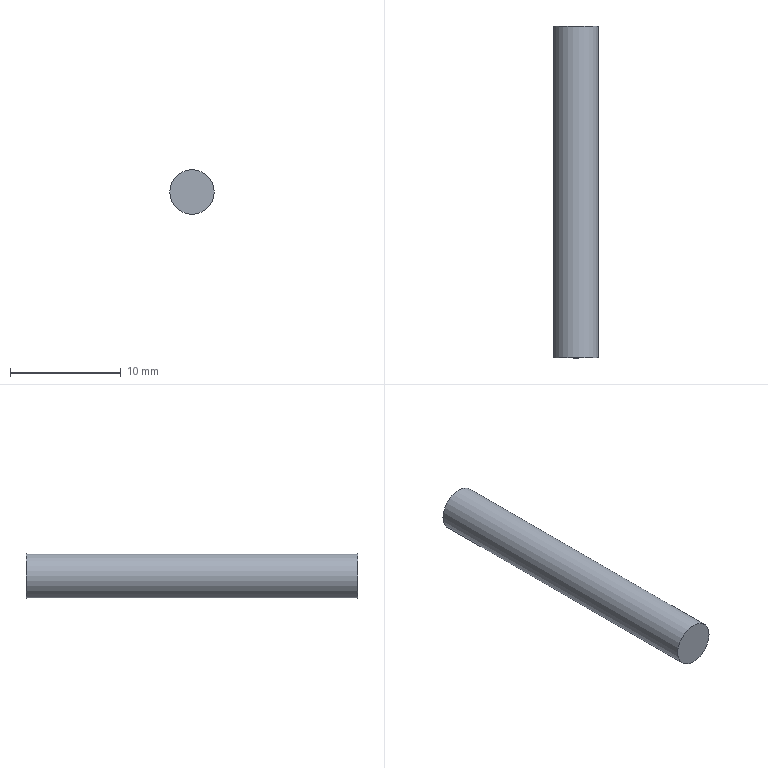Component | NX | STUD_M4 | 1 solid | 3 faces | box 4.01 x 30 x 4.01 mm | volume 379 mm3 | plane 2 | cylinder 1 | commonest cylinder face diameters 4.013 x1
STEP:
#1=CARTESIAN_POINT('',(0.,0.,0.));
#2=DIRECTION('',(0.,0.,1.));
#3=DIRECTION('',(1.,0.,0.));
#4=AXIS2_PLACEMENT_3D('',#1,#2,#3);
#5=CARTESIAN_POINT('',(-9.993,32.5,129.5));
#6=VERTEX_POINT('',#5);
#7=CARTESIAN_POINT('',(-12.,32.5,129.5));
#8=DIRECTION('',(0.,-1.,0.));
#9=DIRECTION('',(1.,0.,0.));
#10=AXIS2_PLACEMENT_3D('',#7,#8,#9);
#11=CIRCLE('',#10,2.007);
#12=CARTESIAN_POINT('',(-12.,32.5,129.5));
#13=DIRECTION('',(0.,1.,0.));
#14=DIRECTION('',(1.,0.,0.));
#15=AXIS2_PLACEMENT_3D('',#12,#13,#14);
#16=PLANE('',#15);
#17=CARTESIAN_POINT('',(2.007,0.));
#18=CARTESIAN_POINT('',(2.007,-3.476));
#19=CARTESIAN_POINT('',(-1.003,-1.738));
#20=CARTESIAN_POINT('',(-4.013,-0.));
#21=CARTESIAN_POINT('',(-1.003,1.738));
#22=CARTESIAN_POINT('',(2.007,3.476));
#23=CARTESIAN_POINT('',(2.007,0.));
#24=(BOUNDED_CURVE()B_SPLINE_CURVE(2,(#17,#18,#19,#20,#21,#22,#23),.UNSPECIFIED.,.T.,.F.)B_SPLINE_CURVE_WITH_KNOTS((1,2,2,2,2,1),(-2.094,0.,2.094,4.189,6.283,8.378),.UNSPECIFIED.)CURVE()GEOMETRIC_REPRESENTATION_ITEM()RATIONAL_B_SPLINE_CURVE((1.,0.5,1.,0.5,1.,0.5,1.))REPRESENTATION_ITEM(''));
#25=(GEOMETRIC_REPRESENTATION_CONTEXT(2)PARAMETRIC_REPRESENTATION_CONTEXT()REPRESENTATION_CONTEXT('',''));
#26=DEFINITIONAL_REPRESENTATION('',(#24),#25);
#27=PCURVE('',#16,#26);
#28=CARTESIAN_POINT('',(-12.,2.5,129.5));
#29=DIRECTION('',(0.,1.,0.));
#30=DIRECTION('',(1.,0.,0.));
#31=AXIS2_PLACEMENT_3D('',#28,#29,#30);
#32=CYLINDRICAL_SURFACE('',#31,2.007);
#33=CARTESIAN_POINT('',(6.283,30.));
#34=DIRECTION('',(-1.,0.));
#35=VECTOR('',#34,1.);
#36=LINE('',#33,#35);
#37=(GEOMETRIC_REPRESENTATION_CONTEXT(2)PARAMETRIC_REPRESENTATION_CONTEXT()REPRESENTATION_CONTEXT('',''));
#38=DEFINITIONAL_REPRESENTATION('',(#36),#37);
#39=PCURVE('',#32,#38);
#40=SURFACE_CURVE('',#11,(#27,#39),.PCURVE_S1.);
#41=EDGE_CURVE('',#6,#6,#40,.T.);
#42=ORIENTED_EDGE('',*,*,#41,.F.);
#43=EDGE_LOOP('',(#42));
#44=FACE_BOUND('',#43,.T.);
#45=ADVANCED_FACE('',(#44),#16,.T.);
#46=CARTESIAN_POINT('',(-9.993,2.5,129.5));
#47=VERTEX_POINT('',#46);
#48=CARTESIAN_POINT('',(-12.,2.5,129.5));
#49=DIRECTION('',(0.,1.,0.));
#50=DIRECTION('',(1.,0.,0.));
#51=AXIS2_PLACEMENT_3D('',#48,#49,#50);
#52=CIRCLE('',#51,2.007);
#53=CARTESIAN_POINT('',(-12.,2.5,129.5));
#54=DIRECTION('',(0.,-1.,0.));
#55=DIRECTION('',(-1.,0.,0.));
#56=AXIS2_PLACEMENT_3D('',#53,#54,#55);
#57=PLANE('',#56);
#58=CARTESIAN_POINT('',(-2.007,0.));
#59=CARTESIAN_POINT('',(-2.007,3.476));
#60=CARTESIAN_POINT('',(1.003,1.738));
#61=CARTESIAN_POINT('',(4.013,0.));
#62=CARTESIAN_POINT('',(1.003,-1.738));
#63=CARTESIAN_POINT('',(-2.007,-3.476));
#64=CARTESIAN_POINT('',(-2.007,0.));
#65=(BOUNDED_CURVE()B_SPLINE_CURVE(2,(#58,#59,#60,#61,#62,#63,#64),.UNSPECIFIED.,.T.,.F.)B_SPLINE_CURVE_WITH_KNOTS((1,2,2,2,2,1),(-2.094,0.,2.094,4.189,6.283,8.378),.UNSPECIFIED.)CURVE()GEOMETRIC_REPRESENTATION_ITEM()RATIONAL_B_SPLINE_CURVE((1.,0.5,1.,0.5,1.,0.5,1.))REPRESENTATION_ITEM(''));
#66=(GEOMETRIC_REPRESENTATION_CONTEXT(2)PARAMETRIC_REPRESENTATION_CONTEXT()REPRESENTATION_CONTEXT('',''));
#67=DEFINITIONAL_REPRESENTATION('',(#65),#66);
#68=PCURVE('',#57,#67);
#69=CARTESIAN_POINT('',(0.,0.));
#70=DIRECTION('',(1.,0.));
#71=VECTOR('',#70,1.);
#72=LINE('',#69,#71);
#73=(GEOMETRIC_REPRESENTATION_CONTEXT(2)PARAMETRIC_REPRESENTATION_CONTEXT()REPRESENTATION_CONTEXT('',''));
#74=DEFINITIONAL_REPRESENTATION('',(#72),#73);
#75=PCURVE('',#32,#74);
#76=SURFACE_CURVE('',#52,(#68,#75),.PCURVE_S1.);
#77=EDGE_CURVE('',#47,#47,#76,.T.);
#78=ORIENTED_EDGE('',*,*,#77,.F.);
#79=EDGE_LOOP('',(#78));
#80=FACE_BOUND('',#79,.T.);
#81=ADVANCED_FACE('',(#80),#57,.T.);
#82=ORIENTED_EDGE('',*,*,#41,.T.);
#83=CARTESIAN_POINT('',(-9.993,2.5,129.5));
#84=CARTESIAN_POINT('',(-9.993,32.5,129.5));
#85=B_SPLINE_CURVE_WITH_KNOTS('',1,(#83,#84),.UNSPECIFIED.,.F.,.F.,(2,2),(0.,30.),.PIECEWISE_BEZIER_KNOTS.);
#86=CARTESIAN_POINT('',(0.,0.));
#87=DIRECTION('',(0.,1.));
#88=VECTOR('',#87,1.);
#89=LINE('',#86,#88);
#90=(GEOMETRIC_REPRESENTATION_CONTEXT(2)PARAMETRIC_REPRESENTATION_CONTEXT()REPRESENTATION_CONTEXT('',''));
#91=DEFINITIONAL_REPRESENTATION('',(#89),#90);
#92=PCURVE('',#32,#91);
#93=CARTESIAN_POINT('',(6.283,0.));
#94=DIRECTION('',(0.,1.));
#95=VECTOR('',#94,1.);
#96=LINE('',#93,#95);
#97=(GEOMETRIC_REPRESENTATION_CONTEXT(2)PARAMETRIC_REPRESENTATION_CONTEXT()REPRESENTATION_CONTEXT('',''));
#98=DEFINITIONAL_REPRESENTATION('',(#96),#97);
#99=PCURVE('',#32,#98);
#100=SEAM_CURVE('',#85,(#92,#99),.PCURVE_S1.);
#101=EDGE_CURVE('',#47,#6,#100,.T.);
#102=ORIENTED_EDGE('',*,*,#101,.F.);
#103=ORIENTED_EDGE('',*,*,#77,.T.);
#104=ORIENTED_EDGE('',*,*,#101,.T.);
#105=EDGE_LOOP('',(#82,#102,#103,#104));
#106=FACE_BOUND('',#105,.T.);
#107=ADVANCED_FACE('',(#106),#32,.T.);
#108=CLOSED_SHELL('',(#45,#81,#107));
#109=MANIFOLD_SOLID_BREP('',#108);
#110=(LENGTH_UNIT()NAMED_UNIT(*)SI_UNIT(.MILLI.,.METRE.));
#111=UNCERTAINTY_MEASURE_WITH_UNIT(LENGTH_MEASURE(0.00001),#110,'','');
#112=(NAMED_UNIT(*)PLANE_ANGLE_UNIT()SI_UNIT($,.RADIAN.));
#113=(NAMED_UNIT(*)SI_UNIT($,.STERADIAN.)SOLID_ANGLE_UNIT());
#114=(GEOMETRIC_REPRESENTATION_CONTEXT(3)GLOBAL_UNCERTAINTY_ASSIGNED_CONTEXT((#111))GLOBAL_UNIT_ASSIGNED_CONTEXT((#110,#112,#113))REPRESENTATION_CONTEXT('',''));
#115=ADVANCED_BREP_SHAPE_REPRESENTATION('',(#4,#109),#114);